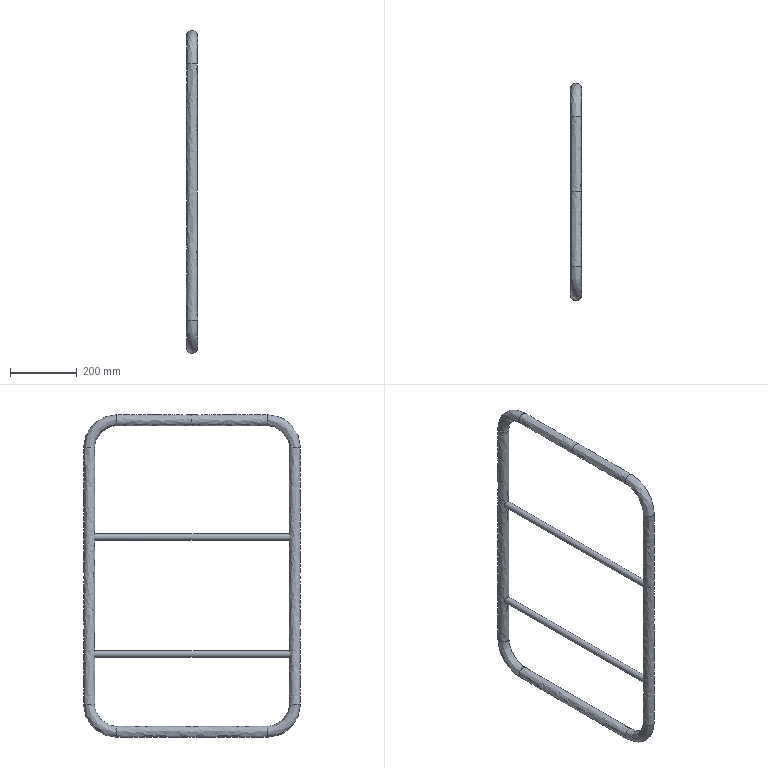Component | NX | 43_5_1_2 | 1 solid | 11 faces | volume 3307811 mm3 | spline 9 | cylinder 2 | commonest cylinder face diameters 20 x2